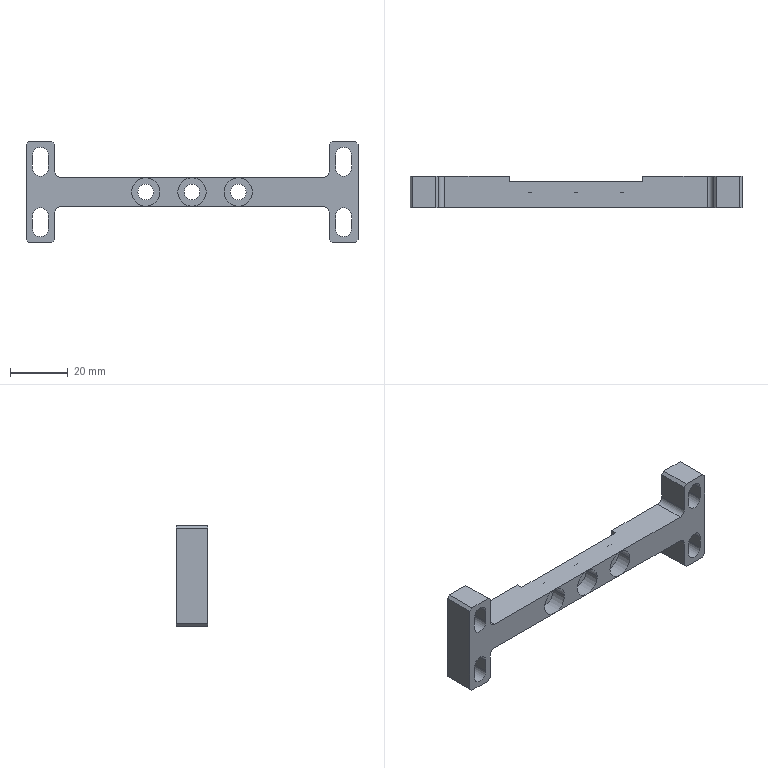Component | SolidWorks | 12-DividingMechanism-1111-1_19-1111-5 | 1 solid | 61 faces | volume 13611 mm3 | plane 37 | cylinder 24 | commonest cylinder face diameters 5.5 x14 9.8 x6 4 x4